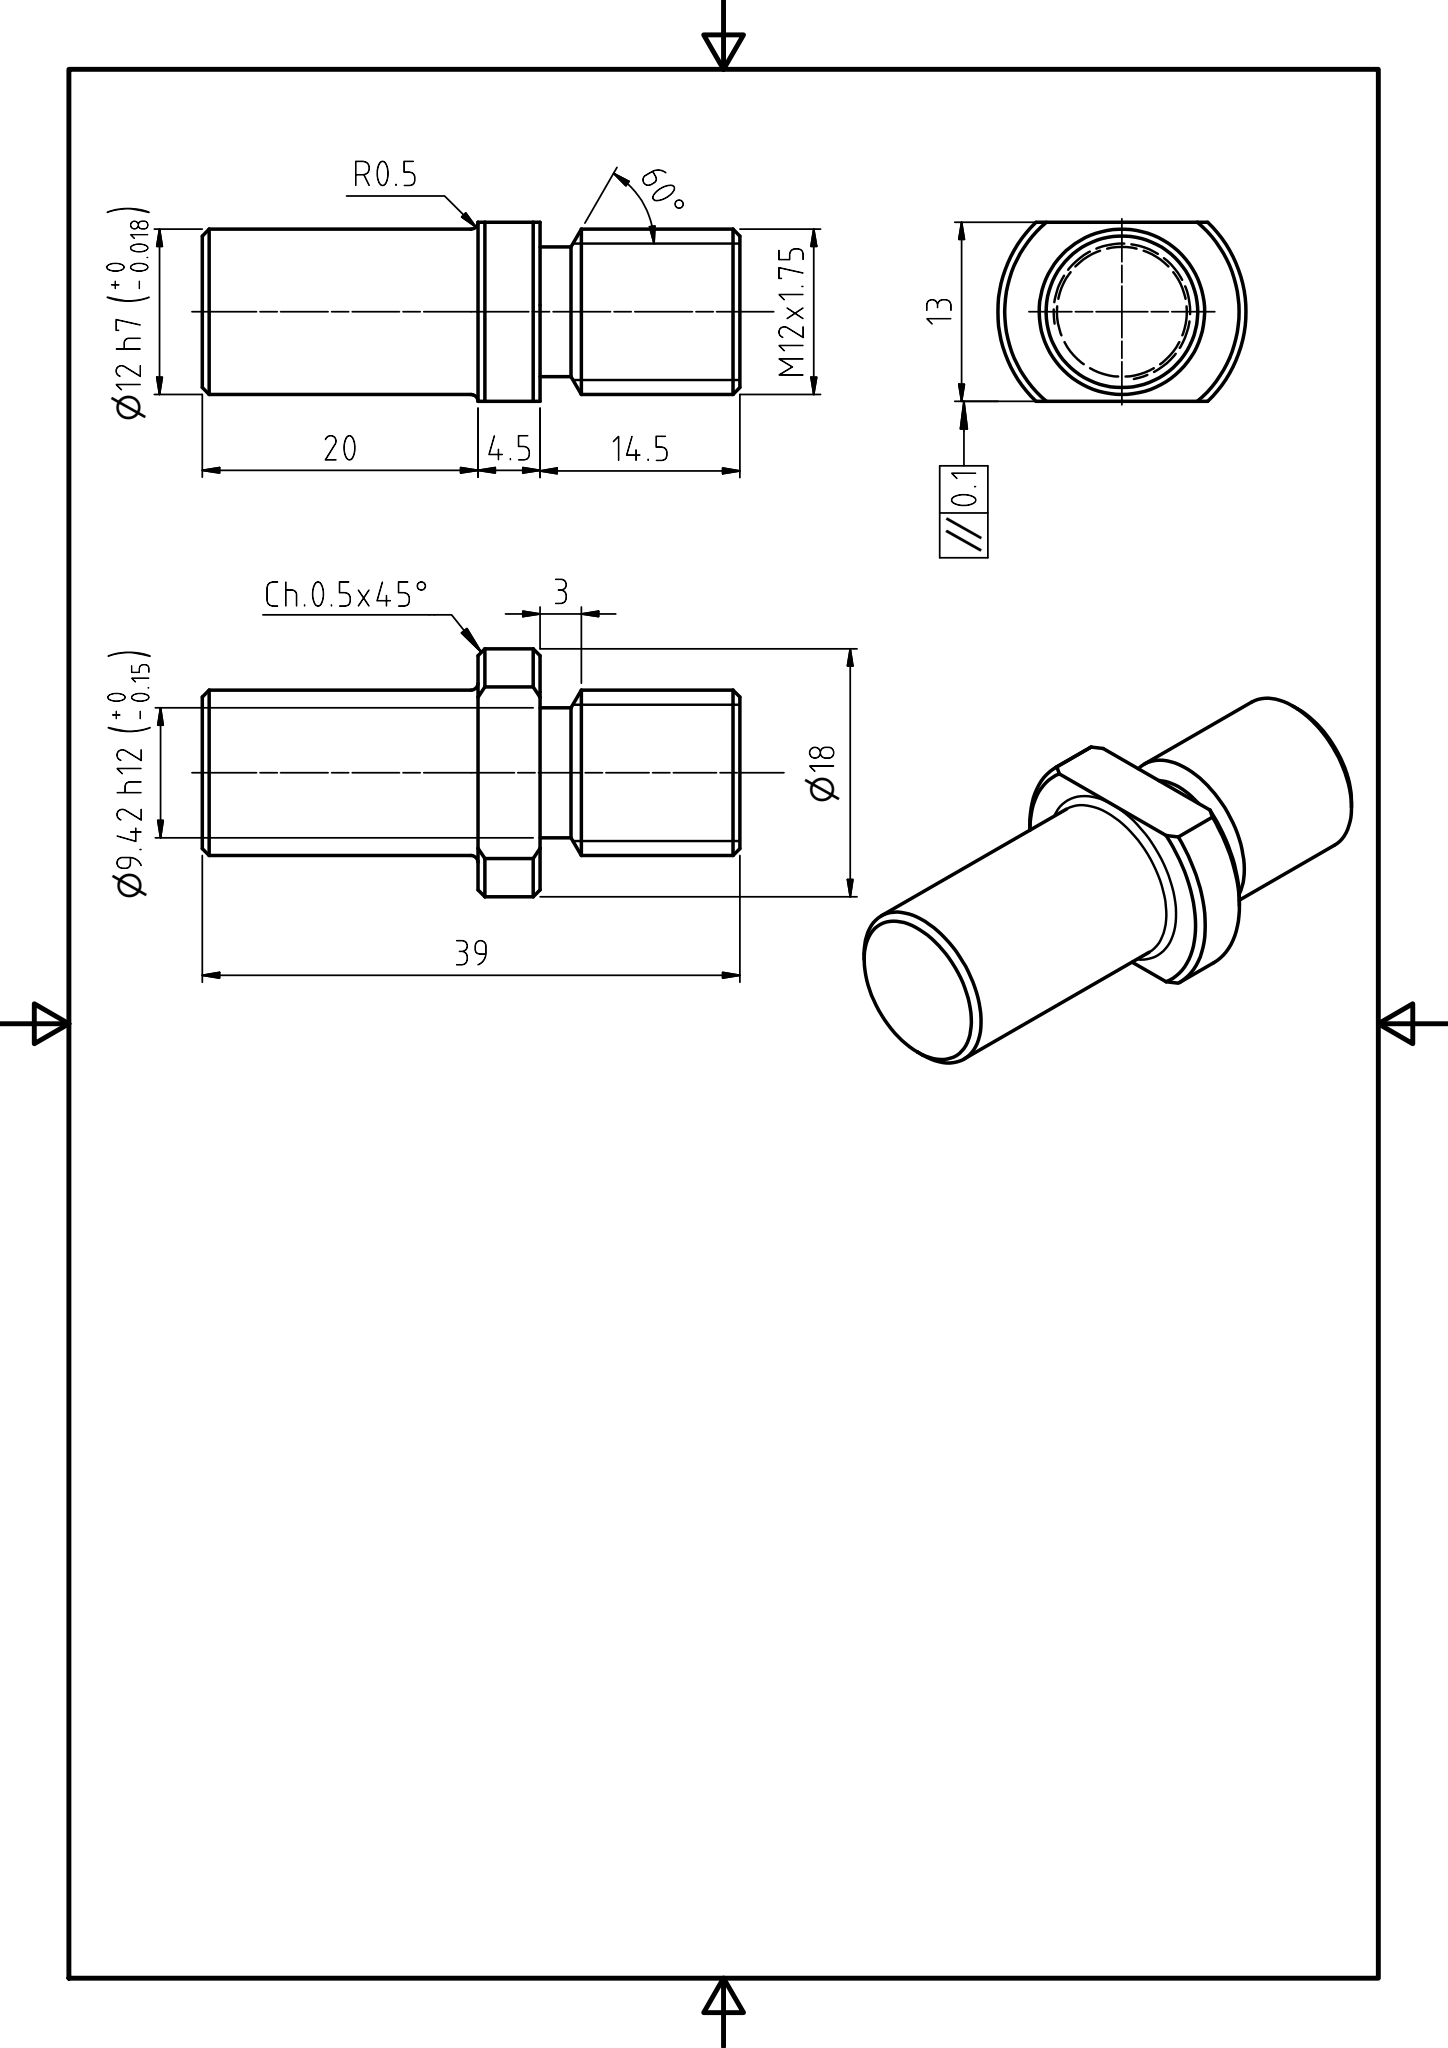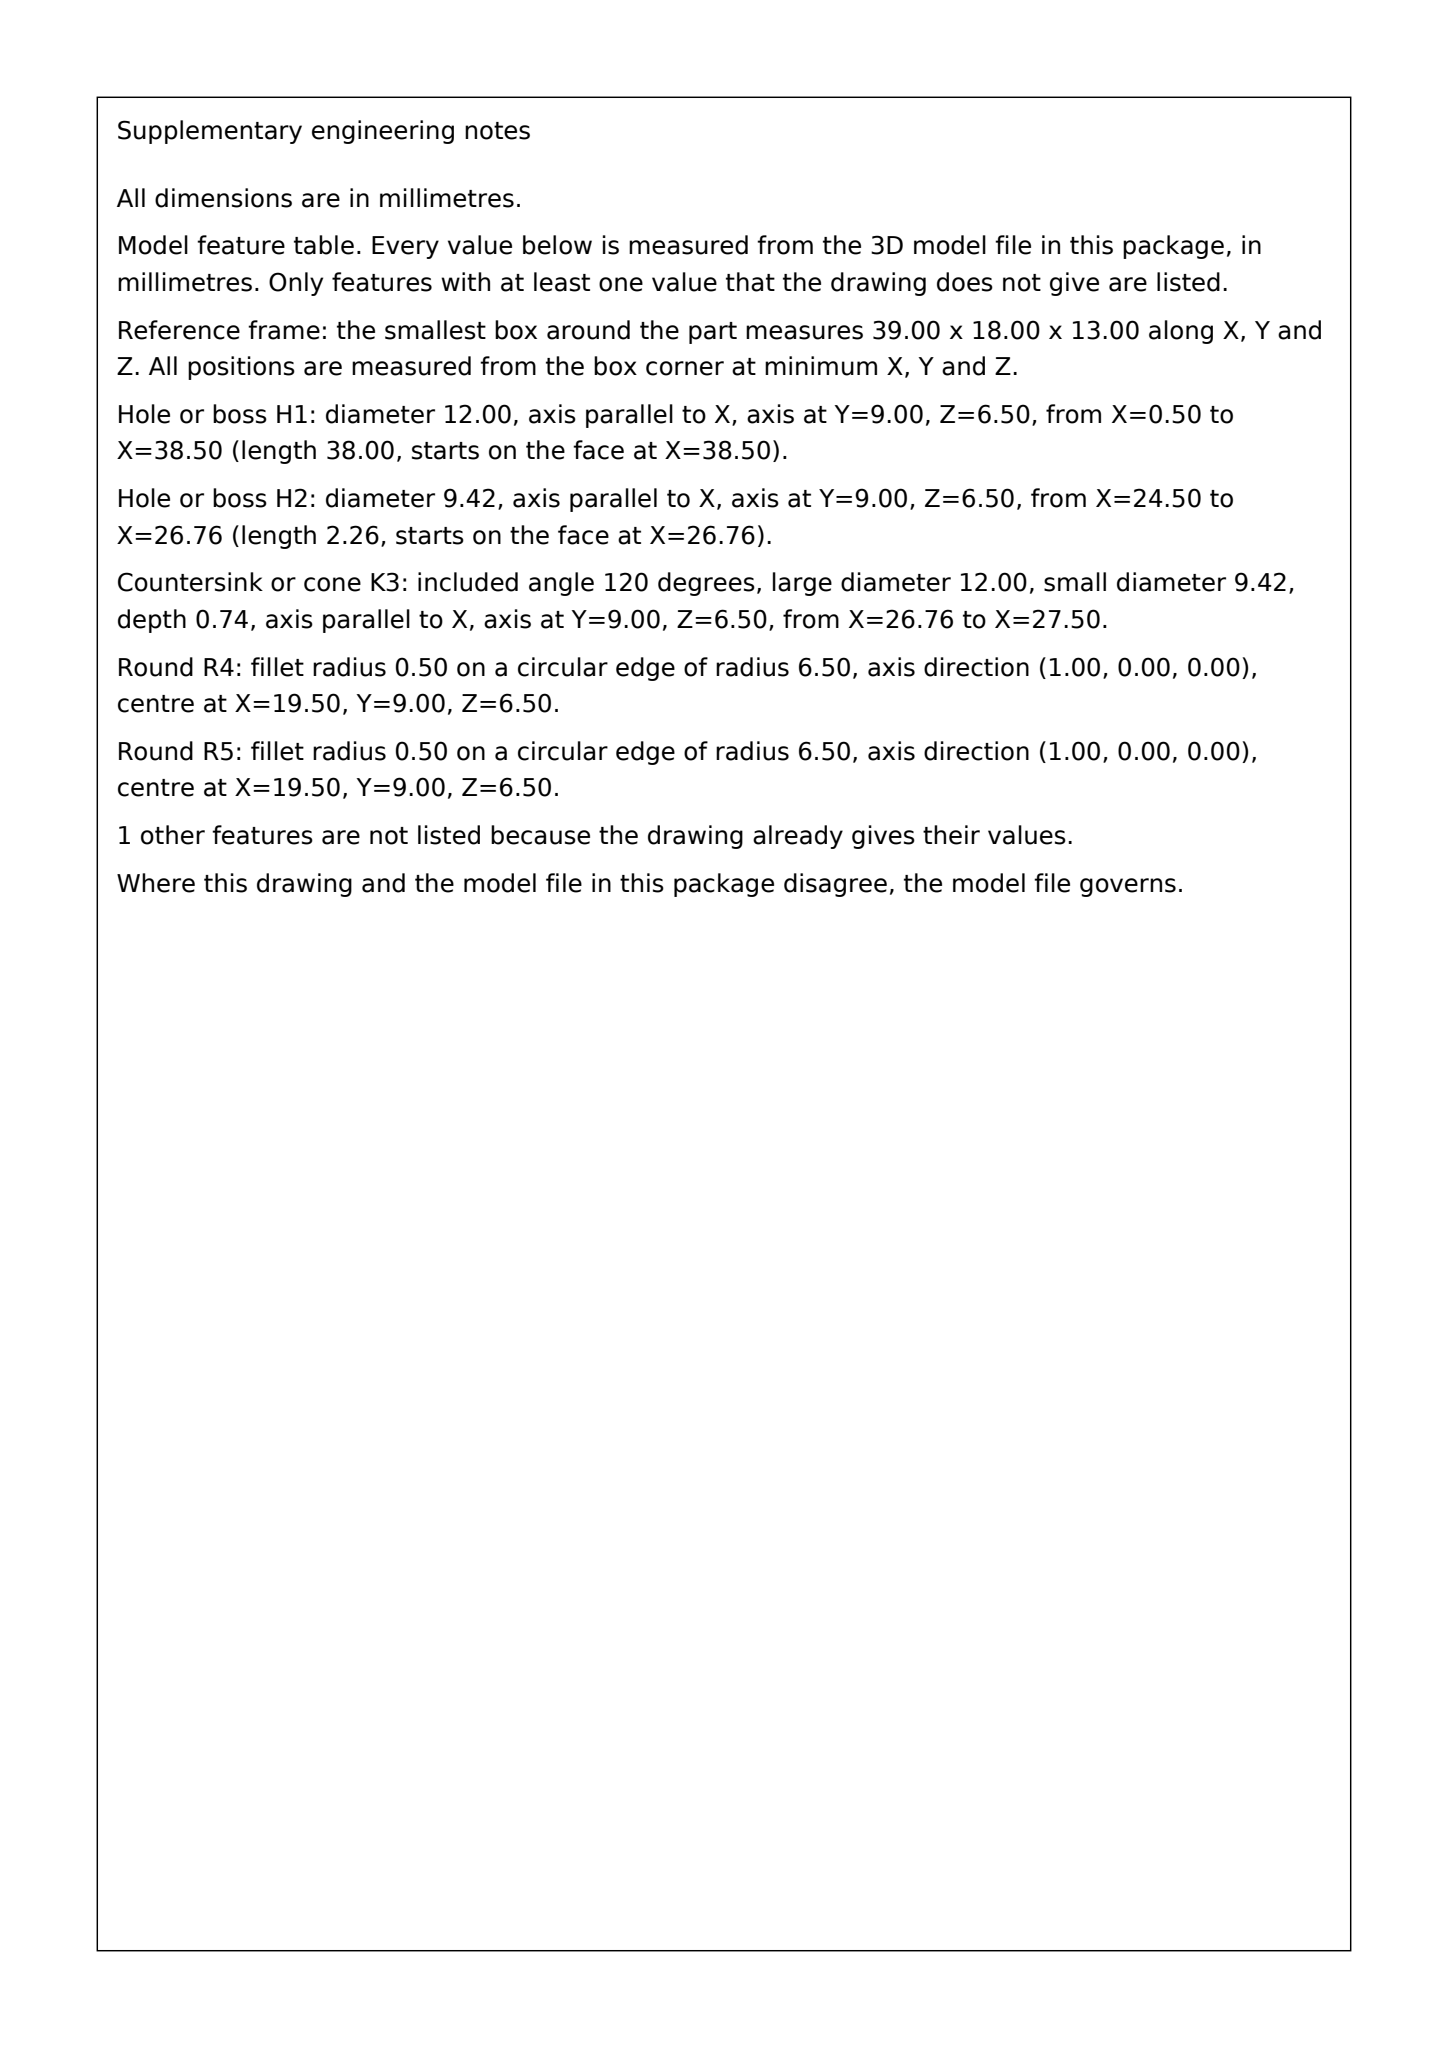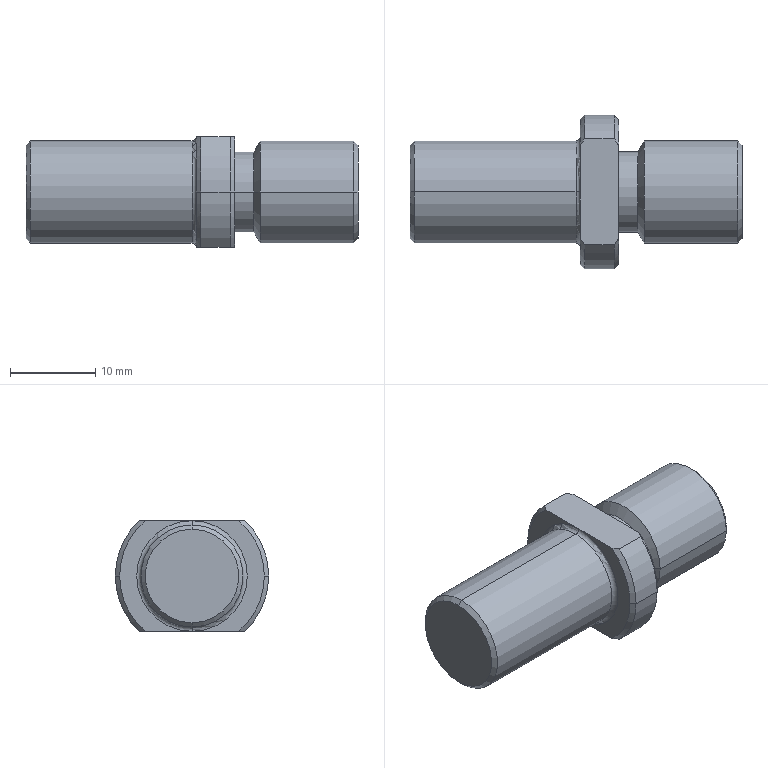Part | SolidWorks | mm | 1 solid | 33 faces | box 39 x 18 x 13 mm | volume 4725 mm3 | cone 14 | cylinder 10 | plane 7 | torus 2 | commonest cylinder face diameters 12 x4 18 x4 9.42 x2